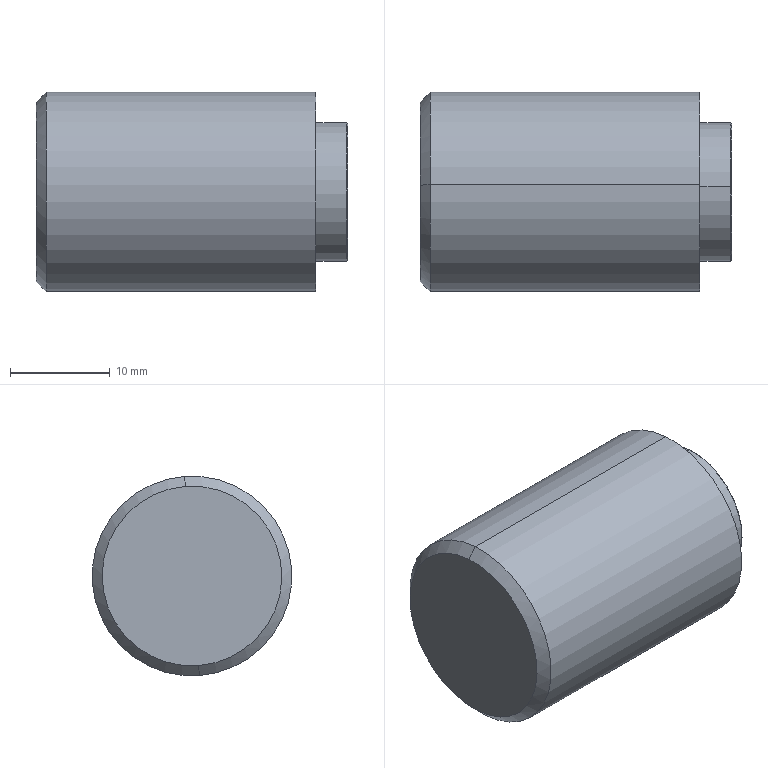Component | SolidWorks | P16BoxWeldment-1_M10WaterproofNutWeldment-10_M10WaterproofStud-1 | 1 solid | 17 faces | box 31.2 x 20 x 20 mm | volume 7158 mm3 | cone 8 | cylinder 6 | plane 3 | commonest cylinder face diameters 10 x2 13.9 x2 20 x2
build123d program:
from build123d import *

# Parameters (mm, degrees)
CHAMFER1_SIZE = 0.3


with BuildPart() as part:
    # Sketch1 → Revolve2 (revolve)
    with BuildSketch(Plane.XY, mode=Mode.PRIVATE) as revolve2_sk:
        Polygon((9.807, 10), (8.807, 9), (8.807, 0), (11.707, 0), (14.207, 5), (40.007, 5), (40.007, 6.85), (39.907, 6.95), (36.807, 6.95), (36.807, 10), align=None)
    revolve(revolve2_sk.sketch.rotate(Axis((0, 0, 0), (1, 0, 0)), 90), axis=Axis((0, 0, 0), (1, 0, 0)))

    # Chamfer1
    chamfer1_edges = [part.edges().sort_by_distance(p)[0] for p in [
        (40.007, 0, -5),
    ]]
    chamfer(chamfer1_edges, length=CHAMFER1_SIZE)


solid = part.part

# Placed as in the assembly
solid = solid.moved(Location((529.849, -186.458, 9.4), (0, 0, 0)))
STEP:
#1=CARTESIAN_POINT('',(22.423,-7.326,0.5664));
#2=VERTEX_POINT('',#1);
#3=CARTESIAN_POINT('',(22.423,-7.355,0.1738));
#4=VERTEX_POINT('',#3);
#5=CARTESIAN_POINT('',(22.423,-7.341,0.3701));
#6=DIRECTION('',(1.,-0.,0.));
#7=DIRECTION('',(0.,0.07403,0.9973));
#8=AXIS2_PLACEMENT_3D('',#5,#6,#7);
#9=CIRCLE('',#8,0.1969);
#10=EDGE_CURVE('',#2,#4,#9,.T.);
#11=ORIENTED_EDGE('',*,*,#10,.F.);
#12=CARTESIAN_POINT('',(22.435,-7.325,0.5782));
#13=VERTEX_POINT('',#12);
#14=CARTESIAN_POINT('',(22.435,-7.325,0.5782));
#15=DIRECTION('',(0.7071,0.05235,0.7052));
#16=VECTOR('',#15,39.37);
#17=LINE('',#14,#16);
#18=EDGE_CURVE('',#2,#13,#17,.T.);
#19=ORIENTED_EDGE('',*,*,#18,.T.);
#20=CARTESIAN_POINT('',(22.435,-7.356,0.162));
#21=VERTEX_POINT('',#20);
#22=CARTESIAN_POINT('',(22.435,-7.341,0.3701));
#23=DIRECTION('',(-1.,0.,-0.));
#24=DIRECTION('',(0.,0.07403,0.9973));
#25=AXIS2_PLACEMENT_3D('',#22,#23,#24);
#26=CIRCLE('',#25,0.2087);
#27=EDGE_CURVE('',#21,#13,#26,.T.);
#28=ORIENTED_EDGE('',*,*,#27,.F.);
#29=CARTESIAN_POINT('',(22.435,-7.356,0.162));
#30=DIRECTION('',(0.7071,-0.05235,-0.7052));
#31=VECTOR('',#30,39.37);
#32=LINE('',#29,#31);
#33=EDGE_CURVE('',#4,#21,#32,.T.);
#34=ORIENTED_EDGE('',*,*,#33,.F.);
#35=EDGE_LOOP('',(#11,#19,#28,#34));
#36=FACE_OUTER_BOUND('',#35,.T.);
#37=CARTESIAN_POINT('',(22.435,-7.341,0.3701));
#38=DIRECTION('',(1.,-0.,0.));
#39=DIRECTION('',(0.,-0.07403,-0.9973));
#40=AXIS2_PLACEMENT_3D('',#37,#38,#39);
#41=CONICAL_SURFACE('',#40,0.2087,0.7854);
#42=ADVANCED_FACE('',(#36),#41,.F.);
#43=CARTESIAN_POINT('',(21.207,-7.315,0.7234));
#44=VERTEX_POINT('',#43);
#45=CARTESIAN_POINT('',(21.207,-7.367,0.01672));
#46=VERTEX_POINT('',#45);
#47=CARTESIAN_POINT('',(21.207,-7.341,0.3701));
#48=DIRECTION('',(-1.,0.,-0.));
#49=DIRECTION('',(0.,0.07403,0.9973));
#50=AXIS2_PLACEMENT_3D('',#47,#48,#49);
#51=CIRCLE('',#50,0.3543);
#52=EDGE_CURVE('',#44,#46,#51,.T.);
#53=ORIENTED_EDGE('',*,*,#52,.F.);
#54=CARTESIAN_POINT('',(21.246,-7.312,0.7627));
#55=VERTEX_POINT('',#54);
#56=CARTESIAN_POINT('',(21.246,-7.312,0.7627));
#57=DIRECTION('',(0.7071,0.05235,0.7052));
#58=VECTOR('',#57,39.37);
#59=LINE('',#56,#58);
#60=EDGE_CURVE('',#44,#55,#59,.T.);
#61=ORIENTED_EDGE('',*,*,#60,.T.);
#62=CARTESIAN_POINT('',(21.246,-7.37,-0.02254));
#63=VERTEX_POINT('',#62);
#64=CARTESIAN_POINT('',(21.246,-7.341,0.3701));
#65=DIRECTION('',(-1.,0.,-0.));
#66=DIRECTION('',(0.,0.07403,0.9973));
#67=AXIS2_PLACEMENT_3D('',#64,#65,#66);
#68=CIRCLE('',#67,0.3937);
#69=EDGE_CURVE('',#55,#63,#68,.T.);
#70=ORIENTED_EDGE('',*,*,#69,.T.);
#71=CARTESIAN_POINT('',(21.246,-7.37,-0.02254));
#72=DIRECTION('',(0.7071,-0.05235,-0.7052));
#73=VECTOR('',#72,39.37);
#74=LINE('',#71,#73);
#75=EDGE_CURVE('',#46,#63,#74,.T.);
#76=ORIENTED_EDGE('',*,*,#75,.F.);
#77=EDGE_LOOP('',(#53,#61,#70,#76));
#78=FACE_OUTER_BOUND('',#77,.T.);
#79=CARTESIAN_POINT('',(21.246,-7.341,0.3701));
#80=DIRECTION('',(1.,-0.,0.));
#81=DIRECTION('',(0.,-0.07403,-0.9973));
#82=AXIS2_PLACEMENT_3D('',#79,#80,#81);
#83=CONICAL_SURFACE('',#82,0.3937,0.7854);
#84=ADVANCED_FACE('',(#78),#83,.T.);
#85=CARTESIAN_POINT('',(21.321,-7.341,0.3701));
#86=VERTEX_POINT('',#85);
#87=CARTESIAN_POINT('',(21.42,-7.355,0.1738));
#88=VERTEX_POINT('',#87);
#89=CARTESIAN_POINT('',(21.321,-7.341,0.3701));
#90=DIRECTION('',(0.4472,-0.06622,-0.892));
#91=VECTOR('',#90,39.37);
#92=LINE('',#89,#91);
#93=EDGE_CURVE('',#86,#88,#92,.T.);
#94=ORIENTED_EDGE('',*,*,#93,.F.);
#95=CARTESIAN_POINT('',(21.42,-7.326,0.5664));
#96=VERTEX_POINT('',#95);
#97=CARTESIAN_POINT('',(21.321,-7.341,0.3701));
#98=DIRECTION('',(0.4472,0.06622,0.892));
#99=VECTOR('',#98,39.37);
#100=LINE('',#97,#99);
#101=EDGE_CURVE('',#86,#96,#100,.T.);
#102=ORIENTED_EDGE('',*,*,#101,.T.);
#103=CARTESIAN_POINT('',(21.42,-7.341,0.3701));
#104=DIRECTION('',(-1.,0.,-0.));
#105=DIRECTION('',(0.,0.07403,0.9973));
#106=AXIS2_PLACEMENT_3D('',#103,#104,#105);
#107=CIRCLE('',#106,0.1969);
#108=EDGE_CURVE('',#88,#96,#107,.T.);
#109=ORIENTED_EDGE('',*,*,#108,.F.);
#110=EDGE_LOOP('',(#94,#102,#109));
#111=FACE_OUTER_BOUND('',#110,.T.);
#112=CARTESIAN_POINT('',(60.691,-7.341,0.3701));
#113=DIRECTION('',(1.,-0.,0.));
#114=DIRECTION('',(0.,-0.07403,-0.9973));
#115=AXIS2_PLACEMENT_3D('',#112,#113,#114);
#116=CONICAL_SURFACE('',#115,78.74,1.107);
#117=ADVANCED_FACE('',(#111),#116,.F.);
#118=ORIENTED_EDGE('',*,*,#10,.T.);
#119=CARTESIAN_POINT('',(20.86,-7.355,0.1738));
#120=DIRECTION('',(-1.,0.,-0.));
#121=VECTOR('',#120,39.37);
#122=LINE('',#119,#121);
#123=EDGE_CURVE('',#4,#88,#122,.T.);
#124=ORIENTED_EDGE('',*,*,#123,.T.);
#125=ORIENTED_EDGE('',*,*,#108,.T.);
#126=CARTESIAN_POINT('',(20.86,-7.326,0.5664));
#127=DIRECTION('',(-1.,0.,-0.));
#128=VECTOR('',#127,39.37);
#129=LINE('',#126,#128);
#130=EDGE_CURVE('',#2,#96,#129,.T.);
#131=ORIENTED_EDGE('',*,*,#130,.F.);
#132=EDGE_LOOP('',(#118,#124,#125,#131));
#133=FACE_OUTER_BOUND('',#132,.T.);
#134=CARTESIAN_POINT('',(20.86,-7.341,0.3701));
#135=DIRECTION('',(-1.,0.,-0.));
#136=DIRECTION('',(0.,0.07403,0.9973));
#137=AXIS2_PLACEMENT_3D('',#134,#135,#136);
#138=CYLINDRICAL_SURFACE('',#137,0.1969);
#139=ADVANCED_FACE('',(#133),#138,.F.);
#140=CARTESIAN_POINT('',(22.435,-7.321,0.639));
#141=VERTEX_POINT('',#140);
#142=CARTESIAN_POINT('',(22.435,-7.361,0.1011));
#143=VERTEX_POINT('',#142);
#144=CARTESIAN_POINT('',(22.435,-7.341,0.3701));
#145=DIRECTION('',(-1.,0.,-0.));
#146=DIRECTION('',(0.,0.07403,0.9973));
#147=AXIS2_PLACEMENT_3D('',#144,#145,#146);
#148=CIRCLE('',#147,0.2697);
#149=EDGE_CURVE('',#141,#143,#148,.T.);
#150=ORIENTED_EDGE('',*,*,#149,.T.);
#151=CARTESIAN_POINT('',(22.431,-7.361,0.09721));
#152=VERTEX_POINT('',#151);
#153=CARTESIAN_POINT('',(22.435,-7.361,0.1011));
#154=DIRECTION('',(-0.7071,-0.05235,-0.7052));
#155=VECTOR('',#154,39.37);
#156=LINE('',#153,#155);
#157=EDGE_CURVE('',#143,#152,#156,.T.);
#158=ORIENTED_EDGE('',*,*,#157,.T.);
#159=CARTESIAN_POINT('',(22.431,-7.321,0.6429));
#160=VERTEX_POINT('',#159);
#161=CARTESIAN_POINT('',(22.431,-7.341,0.3701));
#162=DIRECTION('',(-1.,0.,-0.));
#163=DIRECTION('',(0.,0.07403,0.9973));
#164=AXIS2_PLACEMENT_3D('',#161,#162,#163);
#165=CIRCLE('',#164,0.2736);
#166=EDGE_CURVE('',#160,#152,#165,.T.);
#167=ORIENTED_EDGE('',*,*,#166,.F.);
#168=CARTESIAN_POINT('',(22.435,-7.321,0.639));
#169=DIRECTION('',(-0.7071,0.05235,0.7052));
#170=VECTOR('',#169,39.37);
#171=LINE('',#168,#170);
#172=EDGE_CURVE('',#141,#160,#171,.T.);
#173=ORIENTED_EDGE('',*,*,#172,.F.);
#174=EDGE_LOOP('',(#150,#158,#167,#173));
#175=FACE_OUTER_BOUND('',#174,.T.);
#176=CARTESIAN_POINT('',(22.435,-7.341,0.3701));
#177=DIRECTION('',(-1.,0.,-0.));
#178=DIRECTION('',(0.,0.07403,0.9973));
#179=AXIS2_PLACEMENT_3D('',#176,#177,#178);
#180=CONICAL_SURFACE('',#179,0.2697,0.7854);
#181=ADVANCED_FACE('',(#175),#180,.T.);
#182=ORIENTED_EDGE('',*,*,#166,.T.);
#183=CARTESIAN_POINT('',(22.309,-7.361,0.09721));
#184=VERTEX_POINT('',#183);
#185=CARTESIAN_POINT('',(20.86,-7.361,0.09721));
#186=DIRECTION('',(-1.,0.,-0.));
#187=VECTOR('',#186,39.37);
#188=LINE('',#185,#187);
#189=EDGE_CURVE('',#152,#184,#188,.T.);
#190=ORIENTED_EDGE('',*,*,#189,.T.);
#191=CARTESIAN_POINT('',(22.309,-7.321,0.6429));
#192=VERTEX_POINT('',#191);
#193=CARTESIAN_POINT('',(22.309,-7.341,0.3701));
#194=DIRECTION('',(-1.,0.,-0.));
#195=DIRECTION('',(0.,0.07403,0.9973));
#196=AXIS2_PLACEMENT_3D('',#193,#194,#195);
#197=CIRCLE('',#196,0.2736);
#198=EDGE_CURVE('',#192,#184,#197,.T.);
#199=ORIENTED_EDGE('',*,*,#198,.F.);
#200=CARTESIAN_POINT('',(20.86,-7.321,0.6429));
#201=DIRECTION('',(-1.,0.,-0.));
#202=VECTOR('',#201,39.37);
#203=LINE('',#200,#202);
#204=EDGE_CURVE('',#160,#192,#203,.T.);
#205=ORIENTED_EDGE('',*,*,#204,.F.);
#206=EDGE_LOOP('',(#182,#190,#199,#205));
#207=FACE_OUTER_BOUND('',#206,.T.);
#208=CARTESIAN_POINT('',(20.86,-7.341,0.3701));
#209=DIRECTION('',(-1.,0.,-0.));
#210=DIRECTION('',(0.,0.07403,0.9973));
#211=AXIS2_PLACEMENT_3D('',#208,#209,#210);
#212=CYLINDRICAL_SURFACE('',#211,0.2736);
#213=ADVANCED_FACE('',(#207),#212,.T.);
#214=CARTESIAN_POINT('',(22.309,-7.312,0.7627));
#215=VERTEX_POINT('',#214);
#216=CARTESIAN_POINT('',(22.309,-7.37,-0.02254));
#217=VERTEX_POINT('',#216);
#218=CARTESIAN_POINT('',(22.309,-7.341,0.3701));
#219=DIRECTION('',(-1.,0.,-0.));
#220=DIRECTION('',(0.,0.07403,0.9973));
#221=AXIS2_PLACEMENT_3D('',#218,#219,#220);
#222=CIRCLE('',#221,0.3937);
#223=EDGE_CURVE('',#215,#217,#222,.T.);
#224=ORIENTED_EDGE('',*,*,#223,.T.);
#225=CARTESIAN_POINT('',(20.86,-7.37,-0.02254));
#226=DIRECTION('',(-1.,0.,-0.));
#227=VECTOR('',#226,39.37);
#228=LINE('',#225,#227);
#229=EDGE_CURVE('',#217,#63,#228,.T.);
#230=ORIENTED_EDGE('',*,*,#229,.T.);
#231=ORIENTED_EDGE('',*,*,#69,.F.);
#232=CARTESIAN_POINT('',(20.86,-7.312,0.7627));
#233=DIRECTION('',(-1.,0.,-0.));
#234=VECTOR('',#233,39.37);
#235=LINE('',#232,#234);
#236=EDGE_CURVE('',#215,#55,#235,.T.);
#237=ORIENTED_EDGE('',*,*,#236,.F.);
#238=EDGE_LOOP('',(#224,#230,#231,#237));
#239=FACE_OUTER_BOUND('',#238,.T.);
#240=CARTESIAN_POINT('',(20.86,-7.341,0.3701));
#241=DIRECTION('',(-1.,0.,-0.));
#242=DIRECTION('',(0.,0.07403,0.9973));
#243=AXIS2_PLACEMENT_3D('',#240,#241,#242);
#244=CYLINDRICAL_SURFACE('',#243,0.3937);
#245=ADVANCED_FACE('',(#239),#244,.T.);
#246=ORIENTED_EDGE('',*,*,#229,.F.);
#247=CARTESIAN_POINT('',(22.309,-7.341,0.3701));
#248=DIRECTION('',(-1.,0.,-0.));
#249=DIRECTION('',(0.,0.07403,0.9973));
#250=AXIS2_PLACEMENT_3D('',#247,#248,#249);
#251=CIRCLE('',#250,0.3937);
#252=EDGE_CURVE('',#217,#215,#251,.T.);
#253=ORIENTED_EDGE('',*,*,#252,.T.);
#254=ORIENTED_EDGE('',*,*,#236,.T.);
#255=CARTESIAN_POINT('',(21.246,-7.341,0.3701));
#256=DIRECTION('',(-1.,0.,-0.));
#257=DIRECTION('',(0.,0.07403,0.9973));
#258=AXIS2_PLACEMENT_3D('',#255,#256,#257);
#259=CIRCLE('',#258,0.3937);
#260=EDGE_CURVE('',#63,#55,#259,.T.);
#261=ORIENTED_EDGE('',*,*,#260,.F.);
#262=EDGE_LOOP('',(#246,#253,#254,#261));
#263=FACE_OUTER_BOUND('',#262,.T.);
#264=CARTESIAN_POINT('',(20.86,-7.341,0.3701));
#265=DIRECTION('',(-1.,0.,-0.));
#266=DIRECTION('',(0.,0.07403,0.9973));
#267=AXIS2_PLACEMENT_3D('',#264,#265,#266);
#268=CYLINDRICAL_SURFACE('',#267,0.3937);
#269=ADVANCED_FACE('',(#263),#268,.T.);
#270=ORIENTED_EDGE('',*,*,#223,.F.);
#271=ORIENTED_EDGE('',*,*,#252,.F.);
#272=EDGE_LOOP('',(#270,#271));
#273=FACE_OUTER_BOUND('',#272,.T.);
#274=ORIENTED_EDGE('',*,*,#198,.T.);
#275=CARTESIAN_POINT('',(22.309,-7.341,0.3701));
#276=DIRECTION('',(-1.,0.,-0.));
#277=DIRECTION('',(0.,0.07403,0.9973));
#278=AXIS2_PLACEMENT_3D('',#275,#276,#277);
#279=CIRCLE('',#278,0.2736);
#280=EDGE_CURVE('',#184,#192,#279,.T.);
#281=ORIENTED_EDGE('',*,*,#280,.T.);
#282=EDGE_LOOP('',(#274,#281));
#283=FACE_BOUND('',#282,.T.);
#284=CARTESIAN_POINT('',(22.309,-6.948,0.3409));
#285=DIRECTION('',(-1.,0.,-0.));
#286=DIRECTION('',(-0.,0.07403,0.9973));
#287=AXIS2_PLACEMENT_3D('',#284,#285,#286);
#288=PLANE('',#287);
#289=ADVANCED_FACE('',(#273,#283),#288,.F.);
#290=ORIENTED_EDGE('',*,*,#189,.F.);
#291=CARTESIAN_POINT('',(22.431,-7.341,0.3701));
#292=DIRECTION('',(-1.,0.,-0.));
#293=DIRECTION('',(0.,0.07403,0.9973));
#294=AXIS2_PLACEMENT_3D('',#291,#292,#293);
#295=CIRCLE('',#294,0.2736);
#296=EDGE_CURVE('',#152,#160,#295,.T.);
#297=ORIENTED_EDGE('',*,*,#296,.T.);
#298=ORIENTED_EDGE('',*,*,#204,.T.);
#299=ORIENTED_EDGE('',*,*,#280,.F.);
#300=EDGE_LOOP('',(#290,#297,#298,#299));
#301=FACE_OUTER_BOUND('',#300,.T.);
#302=CARTESIAN_POINT('',(20.86,-7.341,0.3701));
#303=DIRECTION('',(-1.,0.,-0.));
#304=DIRECTION('',(0.,0.07403,0.9973));
#305=AXIS2_PLACEMENT_3D('',#302,#303,#304);
#306=CYLINDRICAL_SURFACE('',#305,0.2736);
#307=ADVANCED_FACE('',(#301),#306,.T.);
#308=ORIENTED_EDGE('',*,*,#157,.F.);
#309=CARTESIAN_POINT('',(22.435,-7.341,0.3701));
#310=DIRECTION('',(-1.,0.,-0.));
#311=DIRECTION('',(0.,0.07403,0.9973));
#312=AXIS2_PLACEMENT_3D('',#309,#310,#311);
#313=CIRCLE('',#312,0.2697);
#314=EDGE_CURVE('',#143,#141,#313,.T.);
#315=ORIENTED_EDGE('',*,*,#314,.T.);
#316=ORIENTED_EDGE('',*,*,#172,.T.);
#317=ORIENTED_EDGE('',*,*,#296,.F.);
#318=EDGE_LOOP('',(#308,#315,#316,#317));
#319=FACE_OUTER_BOUND('',#318,.T.);
#320=CARTESIAN_POINT('',(22.435,-7.341,0.3701));
#321=DIRECTION('',(-1.,0.,-0.));
#322=DIRECTION('',(0.,0.07403,0.9973));
#323=AXIS2_PLACEMENT_3D('',#320,#321,#322);
#324=CONICAL_SURFACE('',#323,0.2697,0.7854);
#325=ADVANCED_FACE('',(#319),#324,.T.);
#326=ORIENTED_EDGE('',*,*,#27,.T.);
#327=CARTESIAN_POINT('',(22.435,-7.341,0.3701));
#328=DIRECTION('',(-1.,0.,-0.));
#329=DIRECTION('',(0.,0.07403,0.9973));
#330=AXIS2_PLACEMENT_3D('',#327,#328,#329);
#331=CIRCLE('',#330,0.2087);
#332=EDGE_CURVE('',#13,#21,#331,.T.);
#333=ORIENTED_EDGE('',*,*,#332,.T.);
#334=EDGE_LOOP('',(#326,#333));
#335=FACE_BOUND('',#334,.T.);
#336=ORIENTED_EDGE('',*,*,#149,.F.);
#337=ORIENTED_EDGE('',*,*,#314,.F.);
#338=EDGE_LOOP('',(#336,#337));
#339=FACE_OUTER_BOUND('',#338,.T.);
#340=CARTESIAN_POINT('',(22.435,-7.072,0.3501));
#341=DIRECTION('',(-1.,0.,-0.));
#342=DIRECTION('',(-0.,0.07403,0.9973));
#343=AXIS2_PLACEMENT_3D('',#340,#341,#342);
#344=PLANE('',#343);
#345=ADVANCED_FACE('',(#335,#339),#344,.F.);
#346=ORIENTED_EDGE('',*,*,#123,.F.);
#347=CARTESIAN_POINT('',(22.423,-7.341,0.3701));
#348=DIRECTION('',(1.,-0.,0.));
#349=DIRECTION('',(0.,0.07403,0.9973));
#350=AXIS2_PLACEMENT_3D('',#347,#348,#349);
#351=CIRCLE('',#350,0.1969);
#352=EDGE_CURVE('',#4,#2,#351,.T.);
#353=ORIENTED_EDGE('',*,*,#352,.T.);
#354=ORIENTED_EDGE('',*,*,#130,.T.);
#355=CARTESIAN_POINT('',(21.42,-7.341,0.3701));
#356=DIRECTION('',(-1.,0.,-0.));
#357=DIRECTION('',(0.,0.07403,0.9973));
#358=AXIS2_PLACEMENT_3D('',#355,#356,#357);
#359=CIRCLE('',#358,0.1969);
#360=EDGE_CURVE('',#96,#88,#359,.T.);
#361=ORIENTED_EDGE('',*,*,#360,.T.);
#362=EDGE_LOOP('',(#346,#353,#354,#361));
#363=FACE_OUTER_BOUND('',#362,.T.);
#364=CARTESIAN_POINT('',(20.86,-7.341,0.3701));
#365=DIRECTION('',(-1.,0.,-0.));
#366=DIRECTION('',(0.,0.07403,0.9973));
#367=AXIS2_PLACEMENT_3D('',#364,#365,#366);
#368=CYLINDRICAL_SURFACE('',#367,0.1969);
#369=ADVANCED_FACE('',(#363),#368,.F.);
#370=ORIENTED_EDGE('',*,*,#101,.F.);
#371=ORIENTED_EDGE('',*,*,#93,.T.);
#372=ORIENTED_EDGE('',*,*,#360,.F.);
#373=EDGE_LOOP('',(#370,#371,#372));
#374=FACE_OUTER_BOUND('',#373,.T.);
#375=CARTESIAN_POINT('',(60.691,-7.341,0.3701));
#376=DIRECTION('',(1.,-0.,0.));
#377=DIRECTION('',(0.,-0.07403,-0.9973));
#378=AXIS2_PLACEMENT_3D('',#375,#376,#377);
#379=CONICAL_SURFACE('',#378,78.74,1.107);
#380=ADVANCED_FACE('',(#374),#379,.F.);
#381=CARTESIAN_POINT('',(21.207,-7.341,0.3701));
#382=DIRECTION('',(-1.,0.,-0.));
#383=DIRECTION('',(0.,0.07403,0.9973));
#384=AXIS2_PLACEMENT_3D('',#381,#382,#383);
#385=CIRCLE('',#384,0.3543);
#386=EDGE_CURVE('',#46,#44,#385,.T.);
#387=ORIENTED_EDGE('',*,*,#386,.T.);
#388=ORIENTED_EDGE('',*,*,#52,.T.);
#389=EDGE_LOOP('',(#387,#388));
#390=FACE_OUTER_BOUND('',#389,.T.);
#391=CARTESIAN_POINT('',(21.207,-7.341,0.3701));
#392=DIRECTION('',(1.,-0.,0.));
#393=DIRECTION('',(0.,-0.07403,-0.9973));
#394=AXIS2_PLACEMENT_3D('',#391,#392,#393);
#395=PLANE('',#394);
#396=ADVANCED_FACE('',(#390),#395,.F.);
#397=ORIENTED_EDGE('',*,*,#60,.F.);
#398=ORIENTED_EDGE('',*,*,#386,.F.);
#399=ORIENTED_EDGE('',*,*,#75,.T.);
#400=ORIENTED_EDGE('',*,*,#260,.T.);
#401=EDGE_LOOP('',(#397,#398,#399,#400));
#402=FACE_OUTER_BOUND('',#401,.T.);
#403=CARTESIAN_POINT('',(21.246,-7.341,0.3701));
#404=DIRECTION('',(1.,-0.,0.));
#405=DIRECTION('',(0.,-0.07403,-0.9973));
#406=AXIS2_PLACEMENT_3D('',#403,#404,#405);
#407=CONICAL_SURFACE('',#406,0.3937,0.7854);
#408=ADVANCED_FACE('',(#402),#407,.T.);
#409=ORIENTED_EDGE('',*,*,#18,.F.);
#410=ORIENTED_EDGE('',*,*,#352,.F.);
#411=ORIENTED_EDGE('',*,*,#33,.T.);
#412=ORIENTED_EDGE('',*,*,#332,.F.);
#413=EDGE_LOOP('',(#409,#410,#411,#412));
#414=FACE_OUTER_BOUND('',#413,.T.);
#415=CARTESIAN_POINT('',(22.435,-7.341,0.3701));
#416=DIRECTION('',(1.,-0.,0.));
#417=DIRECTION('',(0.,-0.07403,-0.9973));
#418=AXIS2_PLACEMENT_3D('',#415,#416,#417);
#419=CONICAL_SURFACE('',#418,0.2087,0.7854);
#420=ADVANCED_FACE('',(#414),#419,.F.);
#421=CLOSED_SHELL('',(#42,#84,#117,#139,#181,#213,#245,#269,#289,#307,#325,#345,#369,#380,#396,#408,#420));
#422=MANIFOLD_SOLID_BREP('',#421);
#423=CARTESIAN_POINT('',(0.,0.,0.));
#424=DIRECTION('',(0.,0.,1.));
#425=DIRECTION('',(1.,0.,0.));
#426=AXIS2_PLACEMENT_3D('',#423,#424,#425);
#427=(LENGTH_UNIT()NAMED_UNIT(*)SI_UNIT($,.METRE.));
#428=LENGTH_MEASURE_WITH_UNIT(LENGTH_MEASURE(0.0254),#427);
#429=DIMENSIONAL_EXPONENTS(1.,0.,0.,0.,0.,0.,0.);
#430=(CONVERSION_BASED_UNIT('',#428)LENGTH_UNIT()NAMED_UNIT(#429));
#431=UNCERTAINTY_MEASURE_WITH_UNIT(LENGTH_MEASURE(0.00001),#430,'','');
#432=(NAMED_UNIT(*)PLANE_ANGLE_UNIT()SI_UNIT($,.RADIAN.));
#433=(NAMED_UNIT(*)SI_UNIT($,.STERADIAN.)SOLID_ANGLE_UNIT());
#434=(GEOMETRIC_REPRESENTATION_CONTEXT(3)GLOBAL_UNCERTAINTY_ASSIGNED_CONTEXT((#431))GLOBAL_UNIT_ASSIGNED_CONTEXT((#430,#432,#433))REPRESENTATION_CONTEXT('',''));
#435=ADVANCED_BREP_SHAPE_REPRESENTATION('',(#422,#426),#434);
#436=COLOUR_RGB('',0.7922,0.8196,0.9333);
#437=FILL_AREA_STYLE_COLOUR('',#436);
#438=FILL_AREA_STYLE('',(#437));
#439=SURFACE_STYLE_FILL_AREA(#438);
#440=SURFACE_SIDE_STYLE('',(#439));
#441=SURFACE_STYLE_USAGE(.BOTH.,#440);
#442=PRESENTATION_STYLE_ASSIGNMENT((#441));
#443=STYLED_ITEM('',(#442),#422);
#444=PRESENTATION_LAYER_ASSIGNMENT('','',(#443));
#445=(LENGTH_UNIT()NAMED_UNIT(*)SI_UNIT($,.METRE.));
#446=LENGTH_MEASURE_WITH_UNIT(LENGTH_MEASURE(0.0254),#445);
#447=DIMENSIONAL_EXPONENTS(1.,0.,0.,0.,0.,0.,0.);
#448=(CONVERSION_BASED_UNIT('',#446)LENGTH_UNIT()NAMED_UNIT(#447));
#449=UNCERTAINTY_MEASURE_WITH_UNIT(LENGTH_MEASURE(0.00001),#448,'','');
#450=(NAMED_UNIT(*)PLANE_ANGLE_UNIT()SI_UNIT($,.RADIAN.));
#451=(NAMED_UNIT(*)SI_UNIT($,.STERADIAN.)SOLID_ANGLE_UNIT());
#452=(GEOMETRIC_REPRESENTATION_CONTEXT(3)GLOBAL_UNCERTAINTY_ASSIGNED_CONTEXT((#449))GLOBAL_UNIT_ASSIGNED_CONTEXT((#448,#450,#451))REPRESENTATION_CONTEXT('',''));
#453=MECHANICAL_DESIGN_GEOMETRIC_PRESENTATION_REPRESENTATION('',(#443),#452);